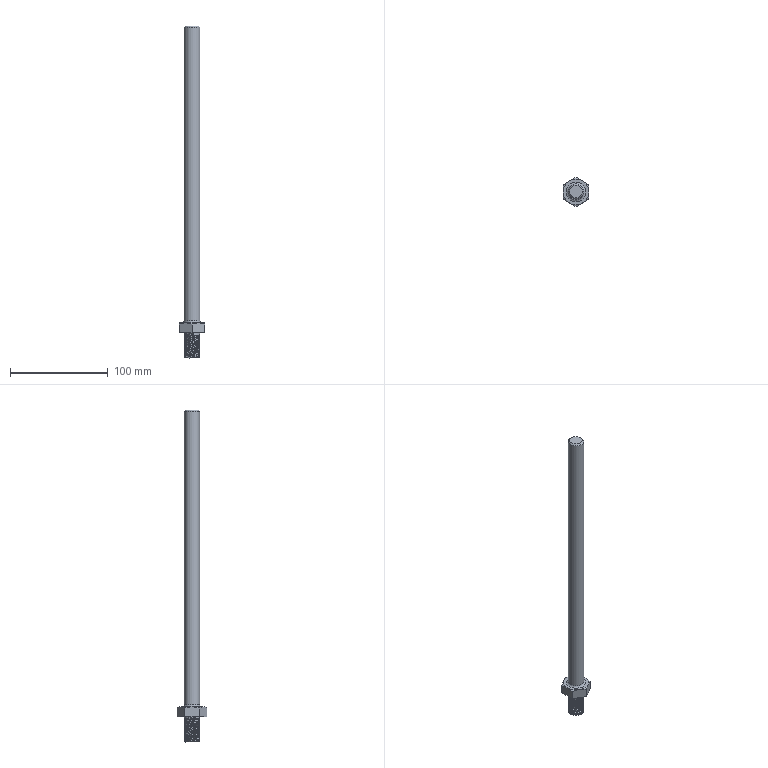Component | NX | 2 | 1 solid | 35 faces | volume 71640 mm3 | cylinder 14 | plane 11 | cone 7 | spline 2 | torus 1 | commonest cylinder face diameters 16 x13 14.7 x1